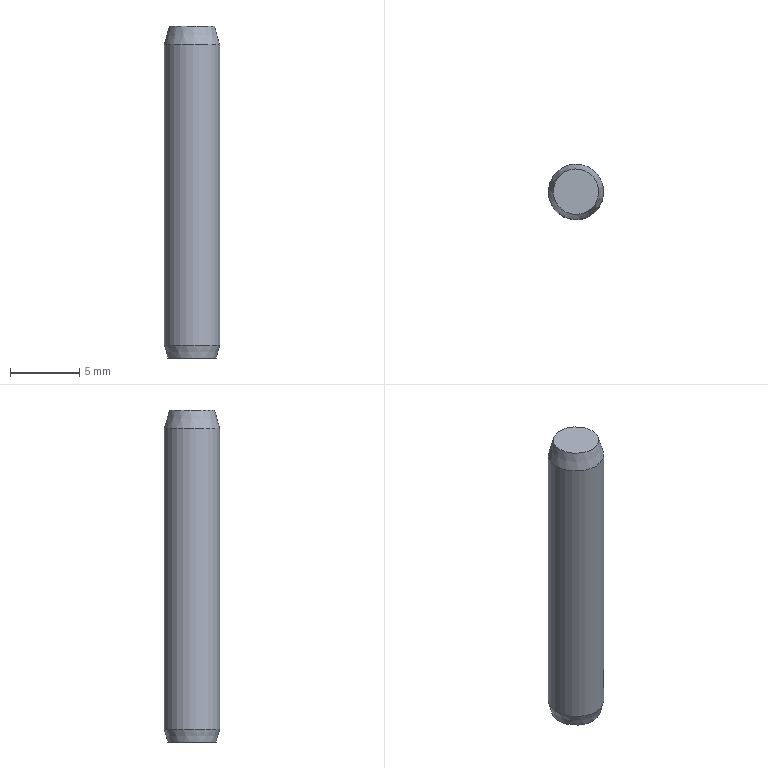Component | NX | 15_T120_1_M4X24_THREADED_DOWEL_PIN_2 | 1 solid | 9 faces | box 4 x 4 x 24 mm | volume 280 mm3 | cone 4 | cylinder 3 | plane 2 | commonest cylinder face diameters 4 x1 1.22 x1 2.3 x1
STEP:
#1=CARTESIAN_POINT('',(0.,0.,0.));
#2=DIRECTION('',(0.,0.,1.));
#3=DIRECTION('',(1.,0.,0.));
#4=AXIS2_PLACEMENT_3D('',#1,#2,#3);
#5=CARTESIAN_POINT('',(19.847,13.766,0.9317));
#6=VERTEX_POINT('',#5);
#7=CARTESIAN_POINT('',(18.,13.,0.9317));
#8=DIRECTION('',(0.,0.,1.));
#9=DIRECTION('',(0.9237,0.383,0.));
#10=AXIS2_PLACEMENT_3D('',#7,#8,#9);
#11=CIRCLE('',#10,2.);
#12=CARTESIAN_POINT('',(18.,13.,0.2588));
#13=DIRECTION('',(0.,0.,1.));
#14=DIRECTION('',(0.9237,0.383,0.));
#15=AXIS2_PLACEMENT_3D('',#12,#13,#14);
#16=CONICAL_SURFACE('',#15,1.82,0.2618);
#17=CARTESIAN_POINT('',(0.,0.6728));
#18=DIRECTION('',(1.,0.));
#19=VECTOR('',#18,1.);
#20=LINE('',#17,#19);
#21=(GEOMETRIC_REPRESENTATION_CONTEXT(2)PARAMETRIC_REPRESENTATION_CONTEXT()REPRESENTATION_CONTEXT('',''));
#22=DEFINITIONAL_REPRESENTATION('',(#20),#21);
#23=PCURVE('',#16,#22);
#24=CARTESIAN_POINT('',(18.,13.,-0.));
#25=DIRECTION('',(0.,0.,1.));
#26=DIRECTION('',(0.9237,0.383,0.));
#27=AXIS2_PLACEMENT_3D('',#24,#25,#26);
#28=CYLINDRICAL_SURFACE('',#27,2.);
#29=CARTESIAN_POINT('',(0.,0.9317));
#30=DIRECTION('',(1.,0.));
#31=VECTOR('',#30,1.);
#32=LINE('',#29,#31);
#33=(GEOMETRIC_REPRESENTATION_CONTEXT(2)PARAMETRIC_REPRESENTATION_CONTEXT()REPRESENTATION_CONTEXT('',''));
#34=DEFINITIONAL_REPRESENTATION('',(#32),#33);
#35=PCURVE('',#28,#34);
#36=SURFACE_CURVE('',#11,(#23,#35),.PCURVE_S1.);
#37=EDGE_CURVE('',#6,#6,#36,.T.);
#38=ORIENTED_EDGE('',*,*,#37,.F.);
#39=CARTESIAN_POINT('',(19.617,13.67,-0.));
#40=VERTEX_POINT('',#39);
#41=CARTESIAN_POINT('',(19.617,13.67,-0.));
#42=CARTESIAN_POINT('',(19.847,13.766,0.9317));
#43=B_SPLINE_CURVE_WITH_KNOTS('',1,(#41,#42),.UNSPECIFIED.,.F.,.F.,(2,2),(-0.2679,0.6966),.PIECEWISE_BEZIER_KNOTS.);
#44=CARTESIAN_POINT('',(0.,0.));
#45=DIRECTION('',(0.,1.));
#46=VECTOR('',#45,1.);
#47=LINE('',#44,#46);
#48=(GEOMETRIC_REPRESENTATION_CONTEXT(2)PARAMETRIC_REPRESENTATION_CONTEXT()REPRESENTATION_CONTEXT('',''));
#49=DEFINITIONAL_REPRESENTATION('',(#47),#48);
#50=PCURVE('',#16,#49);
#51=CARTESIAN_POINT('',(6.283,0.));
#52=DIRECTION('',(0.,1.));
#53=VECTOR('',#52,1.);
#54=LINE('',#51,#53);
#55=(GEOMETRIC_REPRESENTATION_CONTEXT(2)PARAMETRIC_REPRESENTATION_CONTEXT()REPRESENTATION_CONTEXT('',''));
#56=DEFINITIONAL_REPRESENTATION('',(#54),#55);
#57=PCURVE('',#16,#56);
#58=SEAM_CURVE('',#43,(#50,#57),.PCURVE_S1.);
#59=EDGE_CURVE('',#40,#6,#58,.T.);
#60=ORIENTED_EDGE('',*,*,#59,.F.);
#61=CARTESIAN_POINT('',(18.,13.,-0.));
#62=DIRECTION('',(0.,0.,1.));
#63=DIRECTION('',(0.9237,0.383,0.));
#64=AXIS2_PLACEMENT_3D('',#61,#62,#63);
#65=CIRCLE('',#64,1.75);
#66=CARTESIAN_POINT('',(0.,-0.2588));
#67=DIRECTION('',(1.,0.));
#68=VECTOR('',#67,1.);
#69=LINE('',#66,#68);
#70=(GEOMETRIC_REPRESENTATION_CONTEXT(2)PARAMETRIC_REPRESENTATION_CONTEXT()REPRESENTATION_CONTEXT('',''));
#71=DEFINITIONAL_REPRESENTATION('',(#69),#70);
#72=PCURVE('',#16,#71);
#73=CARTESIAN_POINT('',(17.176,14.986,-0.));
#74=DIRECTION('',(0.,0.,1.));
#75=DIRECTION('',(0.9237,0.383,0.));
#76=AXIS2_PLACEMENT_3D('',#73,#74,#75);
#77=PLANE('',#76);
#78=CARTESIAN_POINT('',(0.,-2.15));
#79=DIRECTION('',(1.,-0.));
#80=AXIS2_PLACEMENT_2D('',#78,#79);
#81=CIRCLE('',#80,1.75);
#82=(GEOMETRIC_REPRESENTATION_CONTEXT(2)PARAMETRIC_REPRESENTATION_CONTEXT()REPRESENTATION_CONTEXT('',''));
#83=DEFINITIONAL_REPRESENTATION('',(#81),#82);
#84=PCURVE('',#77,#83);
#85=SURFACE_CURVE('',#65,(#72,#84),.PCURVE_S1.);
#86=EDGE_CURVE('',#40,#40,#85,.T.);
#87=ORIENTED_EDGE('',*,*,#86,.T.);
#88=ORIENTED_EDGE('',*,*,#59,.T.);
#89=EDGE_LOOP('',(#38,#60,#87,#88));
#90=FACE_BOUND('',#89,.T.);
#91=ADVANCED_FACE('',(#90),#16,.T.);
#92=CARTESIAN_POINT('',(19.847,13.766,22.668));
#93=VERTEX_POINT('',#92);
#94=CARTESIAN_POINT('',(16.153,12.234,22.668));
#95=VERTEX_POINT('',#94);
#96=CARTESIAN_POINT('',(18.,13.,22.668));
#97=DIRECTION('',(0.,0.,1.));
#98=DIRECTION('',(-0.9237,-0.383,0.));
#99=AXIS2_PLACEMENT_3D('',#96,#97,#98);
#100=CIRCLE('',#99,2.);
#101=CARTESIAN_POINT('',(-3.142,22.668));
#102=DIRECTION('',(1.,0.));
#103=VECTOR('',#102,1.);
#104=LINE('',#101,#103);
#105=(GEOMETRIC_REPRESENTATION_CONTEXT(2)PARAMETRIC_REPRESENTATION_CONTEXT()REPRESENTATION_CONTEXT('',''));
#106=DEFINITIONAL_REPRESENTATION('',(#104),#105);
#107=PCURVE('',#28,#106);
#108=CARTESIAN_POINT('',(18.,13.,22.541));
#109=DIRECTION('',(0.,0.,-1.));
#110=DIRECTION('',(-0.9237,-0.383,0.));
#111=AXIS2_PLACEMENT_3D('',#108,#109,#110);
#112=CONICAL_SURFACE('',#111,2.034,0.2618);
#113=CARTESIAN_POINT('',(6.283,-0.1272));
#114=DIRECTION('',(-1.,0.));
#115=VECTOR('',#114,1.);
#116=LINE('',#113,#115);
#117=(GEOMETRIC_REPRESENTATION_CONTEXT(2)PARAMETRIC_REPRESENTATION_CONTEXT()REPRESENTATION_CONTEXT('',''));
#118=DEFINITIONAL_REPRESENTATION('',(#116),#117);
#119=PCURVE('',#112,#118);
#120=SURFACE_CURVE('',#100,(#107,#119),.PCURVE_S1.);
#121=EDGE_CURVE('',#93,#95,#120,.T.);
#122=ORIENTED_EDGE('',*,*,#121,.F.);
#123=CARTESIAN_POINT('',(19.847,13.766,0.9317));
#124=CARTESIAN_POINT('',(19.847,13.766,22.668));
#125=B_SPLINE_CURVE_WITH_KNOTS('',1,(#123,#124),.UNSPECIFIED.,.F.,.F.,(2,2),(0.9317,22.668),.PIECEWISE_BEZIER_KNOTS.);
#126=CARTESIAN_POINT('',(0.,0.));
#127=DIRECTION('',(0.,1.));
#128=VECTOR('',#127,1.);
#129=LINE('',#126,#128);
#130=(GEOMETRIC_REPRESENTATION_CONTEXT(2)PARAMETRIC_REPRESENTATION_CONTEXT()REPRESENTATION_CONTEXT('',''));
#131=DEFINITIONAL_REPRESENTATION('',(#129),#130);
#132=PCURVE('',#28,#131);
#133=CARTESIAN_POINT('',(6.283,0.));
#134=DIRECTION('',(0.,1.));
#135=VECTOR('',#134,1.);
#136=LINE('',#133,#135);
#137=(GEOMETRIC_REPRESENTATION_CONTEXT(2)PARAMETRIC_REPRESENTATION_CONTEXT()REPRESENTATION_CONTEXT('',''));
#138=DEFINITIONAL_REPRESENTATION('',(#136),#137);
#139=PCURVE('',#28,#138);
#140=SEAM_CURVE('',#125,(#132,#139),.PCURVE_S1.);
#141=EDGE_CURVE('',#6,#93,#140,.T.);
#142=ORIENTED_EDGE('',*,*,#141,.F.);
#143=ORIENTED_EDGE('',*,*,#37,.T.);
#144=ORIENTED_EDGE('',*,*,#141,.T.);
#145=CARTESIAN_POINT('',(18.,13.,22.668));
#146=DIRECTION('',(0.,0.,1.));
#147=DIRECTION('',(-0.9237,-0.383,0.));
#148=AXIS2_PLACEMENT_3D('',#145,#146,#147);
#149=CIRCLE('',#148,2.);
#150=CARTESIAN_POINT('',(3.142,22.668));
#151=DIRECTION('',(1.,0.));
#152=VECTOR('',#151,1.);
#153=LINE('',#150,#152);
#154=(GEOMETRIC_REPRESENTATION_CONTEXT(2)PARAMETRIC_REPRESENTATION_CONTEXT()REPRESENTATION_CONTEXT('',''));
#155=DEFINITIONAL_REPRESENTATION('',(#153),#154);
#156=PCURVE('',#28,#155);
#157=CARTESIAN_POINT('',(6.283,-0.1272));
#158=DIRECTION('',(-1.,0.));
#159=VECTOR('',#158,1.);
#160=LINE('',#157,#159);
#161=(GEOMETRIC_REPRESENTATION_CONTEXT(2)PARAMETRIC_REPRESENTATION_CONTEXT()REPRESENTATION_CONTEXT('',''));
#162=DEFINITIONAL_REPRESENTATION('',(#160),#161);
#163=PCURVE('',#112,#162);
#164=SURFACE_CURVE('',#149,(#156,#163),.PCURVE_S1.);
#165=EDGE_CURVE('',#95,#93,#164,.T.);
#166=ORIENTED_EDGE('',*,*,#165,.F.);
#167=EDGE_LOOP('',(#122,#142,#143,#144,#166));
#168=FACE_BOUND('',#167,.T.);
#169=ADVANCED_FACE('',(#168),#28,.T.);
#170=CARTESIAN_POINT('',(16.482,12.371,24.));
#171=VERTEX_POINT('',#170);
#172=CARTESIAN_POINT('',(18.,13.,24.));
#173=DIRECTION('',(0.,0.,1.));
#174=DIRECTION('',(-0.9237,-0.383,0.));
#175=AXIS2_PLACEMENT_3D('',#172,#173,#174);
#176=CIRCLE('',#175,1.643);
#177=CARTESIAN_POINT('',(6.283,-1.459));
#178=DIRECTION('',(-1.,0.));
#179=VECTOR('',#178,1.);
#180=LINE('',#177,#179);
#181=(GEOMETRIC_REPRESENTATION_CONTEXT(2)PARAMETRIC_REPRESENTATION_CONTEXT()REPRESENTATION_CONTEXT('',''));
#182=DEFINITIONAL_REPRESENTATION('',(#180),#181);
#183=PCURVE('',#112,#182);
#184=CARTESIAN_POINT('',(16.974,15.474,24.));
#185=DIRECTION('',(0.,0.,-1.));
#186=DIRECTION('',(-0.9237,-0.383,0.));
#187=AXIS2_PLACEMENT_3D('',#184,#185,#186);
#188=PLANE('',#187);
#189=CARTESIAN_POINT('',(1.643,-2.678));
#190=CARTESIAN_POINT('',(1.643,-5.525));
#191=CARTESIAN_POINT('',(-0.8216,-4.102));
#192=CARTESIAN_POINT('',(-3.286,-2.678));
#193=CARTESIAN_POINT('',(-0.8216,-1.255));
#194=CARTESIAN_POINT('',(1.643,0.1676));
#195=CARTESIAN_POINT('',(1.643,-2.678));
#196=(BOUNDED_CURVE()B_SPLINE_CURVE(2,(#189,#190,#191,#192,#193,#194,#195),.UNSPECIFIED.,.T.,.F.)B_SPLINE_CURVE_WITH_KNOTS((1,2,2,2,2,1),(-2.094,0.,2.094,4.189,6.283,8.378),.UNSPECIFIED.)CURVE()GEOMETRIC_REPRESENTATION_ITEM()RATIONAL_B_SPLINE_CURVE((1.,0.5,1.,0.5,1.,0.5,1.))REPRESENTATION_ITEM(''));
#197=(GEOMETRIC_REPRESENTATION_CONTEXT(2)PARAMETRIC_REPRESENTATION_CONTEXT()REPRESENTATION_CONTEXT('',''));
#198=DEFINITIONAL_REPRESENTATION('',(#196),#197);
#199=PCURVE('',#188,#198);
#200=SURFACE_CURVE('',#176,(#183,#199),.PCURVE_S1.);
#201=EDGE_CURVE('',#171,#171,#200,.T.);
#202=ORIENTED_EDGE('',*,*,#201,.F.);
#203=CARTESIAN_POINT('',(16.482,12.371,24.));
#204=CARTESIAN_POINT('',(16.153,12.234,22.668));
#205=B_SPLINE_CURVE_WITH_KNOTS('',1,(#203,#204),.UNSPECIFIED.,.F.,.F.,(2,2),(-1.51,-0.1317),.PIECEWISE_BEZIER_KNOTS.);
#206=CARTESIAN_POINT('',(6.283,0.));
#207=DIRECTION('',(0.,1.));
#208=VECTOR('',#207,1.);
#209=LINE('',#206,#208);
#210=(GEOMETRIC_REPRESENTATION_CONTEXT(2)PARAMETRIC_REPRESENTATION_CONTEXT()REPRESENTATION_CONTEXT('',''));
#211=DEFINITIONAL_REPRESENTATION('',(#209),#210);
#212=PCURVE('',#112,#211);
#213=CARTESIAN_POINT('',(0.,0.));
#214=DIRECTION('',(0.,1.));
#215=VECTOR('',#214,1.);
#216=LINE('',#213,#215);
#217=(GEOMETRIC_REPRESENTATION_CONTEXT(2)PARAMETRIC_REPRESENTATION_CONTEXT()REPRESENTATION_CONTEXT('',''));
#218=DEFINITIONAL_REPRESENTATION('',(#216),#217);
#219=PCURVE('',#112,#218);
#220=SEAM_CURVE('',#205,(#212,#219),.PCURVE_S1.);
#221=EDGE_CURVE('',#171,#95,#220,.T.);
#222=ORIENTED_EDGE('',*,*,#221,.T.);
#223=ORIENTED_EDGE('',*,*,#165,.T.);
#224=ORIENTED_EDGE('',*,*,#121,.T.);
#225=ORIENTED_EDGE('',*,*,#221,.F.);
#226=EDGE_LOOP('',(#202,#222,#223,#224,#225));
#227=FACE_BOUND('',#226,.T.);
#228=ADVANCED_FACE('',(#227),#112,.T.);
#229=ORIENTED_EDGE('',*,*,#201,.T.);
#230=EDGE_LOOP('',(#229));
#231=FACE_BOUND('',#230,.T.);
#232=ADVANCED_FACE('',(#231),#188,.F.);
#233=CARTESIAN_POINT('',(17.437,12.766,10.577));
#234=VERTEX_POINT('',#233);
#235=CARTESIAN_POINT('',(18.,13.,10.577));
#236=DIRECTION('',(0.,0.,1.));
#237=DIRECTION('',(-0.9237,-0.383,0.));
#238=AXIS2_PLACEMENT_3D('',#235,#236,#237);
#239=CIRCLE('',#238,0.61);
#240=CARTESIAN_POINT('',(18.,13.,10.93));
#241=DIRECTION('',(0.,0.,-1.));
#242=DIRECTION('',(-0.9237,-0.383,0.));
#243=AXIS2_PLACEMENT_3D('',#240,#241,#242);
#244=CONICAL_SURFACE('',#243,0.,1.047);
#245=CARTESIAN_POINT('',(6.283,0.3522));
#246=DIRECTION('',(-1.,-0.));
#247=VECTOR('',#246,1.);
#248=LINE('',#245,#247);
#249=(GEOMETRIC_REPRESENTATION_CONTEXT(2)PARAMETRIC_REPRESENTATION_CONTEXT()REPRESENTATION_CONTEXT('',''));
#250=DEFINITIONAL_REPRESENTATION('',(#248),#249);
#251=PCURVE('',#244,#250);
#252=CARTESIAN_POINT('',(18.,13.,-0.));
#253=DIRECTION('',(0.,0.,1.));
#254=DIRECTION('',(0.9237,0.383,0.));
#255=AXIS2_PLACEMENT_3D('',#252,#253,#254);
#256=CYLINDRICAL_SURFACE('',#255,0.61);
#257=CARTESIAN_POINT('',(3.142,10.577));
#258=DIRECTION('',(1.,0.));
#259=VECTOR('',#258,1.);
#260=LINE('',#257,#259);
#261=(GEOMETRIC_REPRESENTATION_CONTEXT(2)PARAMETRIC_REPRESENTATION_CONTEXT()REPRESENTATION_CONTEXT('',''));
#262=DEFINITIONAL_REPRESENTATION('',(#260),#261);
#263=PCURVE('',#256,#262);
#264=SURFACE_CURVE('',#239,(#251,#263),.PCURVE_S1.);
#265=EDGE_CURVE('',#234,#234,#264,.T.);
#266=ORIENTED_EDGE('',*,*,#265,.T.);
#267=CARTESIAN_POINT('',(18.,13.,10.93));
#268=VERTEX_POINT('',#267);
#269=CARTESIAN_POINT('',(18.,13.,10.93));
#270=CARTESIAN_POINT('',(17.437,12.766,10.577));
#271=B_SPLINE_CURVE_WITH_KNOTS('',1,(#269,#270),.UNSPECIFIED.,.F.,.F.,(2,2),(-0.,0.7044),.PIECEWISE_BEZIER_KNOTS.);
#272=CARTESIAN_POINT('',(0.,0.));
#273=DIRECTION('',(0.,1.));
#274=VECTOR('',#273,1.);
#275=LINE('',#272,#274);
#276=(GEOMETRIC_REPRESENTATION_CONTEXT(2)PARAMETRIC_REPRESENTATION_CONTEXT()REPRESENTATION_CONTEXT('',''));
#277=DEFINITIONAL_REPRESENTATION('',(#275),#276);
#278=PCURVE('',#244,#277);
#279=CARTESIAN_POINT('',(6.283,0.));
#280=DIRECTION('',(0.,1.));
#281=VECTOR('',#280,1.);
#282=LINE('',#279,#281);
#283=(GEOMETRIC_REPRESENTATION_CONTEXT(2)PARAMETRIC_REPRESENTATION_CONTEXT()REPRESENTATION_CONTEXT('',''));
#284=DEFINITIONAL_REPRESENTATION('',(#282),#283);
#285=PCURVE('',#244,#284);
#286=SEAM_CURVE('',#271,(#278,#285),.PCURVE_S1.);
#287=EDGE_CURVE('',#268,#234,#286,.T.);
#288=ORIENTED_EDGE('',*,*,#287,.F.);
#289=ORIENTED_EDGE('',*,*,#287,.T.);
#290=EDGE_LOOP('',(#266,#288,#289));
#291=FACE_BOUND('',#290,.F.);
#292=ADVANCED_FACE('',(#291),#244,.F.);
#293=CARTESIAN_POINT('',(17.437,12.766,1.889));
#294=VERTEX_POINT('',#293);
#295=CARTESIAN_POINT('',(18.,13.,1.889));
#296=DIRECTION('',(0.,0.,1.));
#297=DIRECTION('',(-0.9237,-0.383,0.));
#298=AXIS2_PLACEMENT_3D('',#295,#296,#297);
#299=CIRCLE('',#298,0.61);
#300=CARTESIAN_POINT('',(3.142,1.889));
#301=DIRECTION('',(1.,0.));
#302=VECTOR('',#301,1.);
#303=LINE('',#300,#302);
#304=(GEOMETRIC_REPRESENTATION_CONTEXT(2)PARAMETRIC_REPRESENTATION_CONTEXT()REPRESENTATION_CONTEXT('',''));
#305=DEFINITIONAL_REPRESENTATION('',(#303),#304);
#306=PCURVE('',#256,#305);
#307=CARTESIAN_POINT('',(18.,13.,1.312));
#308=DIRECTION('',(0.,0.,-1.));
#309=DIRECTION('',(-0.9237,-0.383,0.));
#310=AXIS2_PLACEMENT_3D('',#307,#308,#309);
#311=CONICAL_SURFACE('',#310,1.61,1.047);
#312=CARTESIAN_POINT('',(6.283,-0.5774));
#313=DIRECTION('',(-1.,0.));
#314=VECTOR('',#313,1.);
#315=LINE('',#312,#314);
#316=(GEOMETRIC_REPRESENTATION_CONTEXT(2)PARAMETRIC_REPRESENTATION_CONTEXT()REPRESENTATION_CONTEXT('',''));
#317=DEFINITIONAL_REPRESENTATION('',(#315),#316);
#318=PCURVE('',#311,#317);
#319=SURFACE_CURVE('',#299,(#306,#318),.PCURVE_S1.);
#320=EDGE_CURVE('',#294,#294,#319,.T.);
#321=ORIENTED_EDGE('',*,*,#320,.T.);
#322=CARTESIAN_POINT('',(17.437,12.766,1.889));
#323=CARTESIAN_POINT('',(17.437,12.766,10.577));
#324=B_SPLINE_CURVE_WITH_KNOTS('',1,(#322,#323),.UNSPECIFIED.,.F.,.F.,(2,2),(1.889,10.577),.PIECEWISE_BEZIER_KNOTS.);
#325=CARTESIAN_POINT('',(9.425,0.));
#326=DIRECTION('',(0.,1.));
#327=VECTOR('',#326,1.);
#328=LINE('',#325,#327);
#329=(GEOMETRIC_REPRESENTATION_CONTEXT(2)PARAMETRIC_REPRESENTATION_CONTEXT()REPRESENTATION_CONTEXT('',''));
#330=DEFINITIONAL_REPRESENTATION('',(#328),#329);
#331=PCURVE('',#256,#330);
#332=CARTESIAN_POINT('',(3.142,0.));
#333=DIRECTION('',(0.,1.));
#334=VECTOR('',#333,1.);
#335=LINE('',#332,#334);
#336=(GEOMETRIC_REPRESENTATION_CONTEXT(2)PARAMETRIC_REPRESENTATION_CONTEXT()REPRESENTATION_CONTEXT('',''));
#337=DEFINITIONAL_REPRESENTATION('',(#335),#336);
#338=PCURVE('',#256,#337);
#339=SEAM_CURVE('',#324,(#331,#338),.PCURVE_S1.);
#340=EDGE_CURVE('',#294,#234,#339,.T.);
#341=ORIENTED_EDGE('',*,*,#340,.T.);
#342=ORIENTED_EDGE('',*,*,#265,.F.);
#343=ORIENTED_EDGE('',*,*,#340,.F.);
#344=EDGE_LOOP('',(#321,#341,#342,#343));
#345=FACE_BOUND('',#344,.F.);
#346=ADVANCED_FACE('',(#345),#256,.F.);
#347=CARTESIAN_POINT('',(16.938,12.559,1.577));
#348=VERTEX_POINT('',#347);
#349=CARTESIAN_POINT('',(19.062,13.441,1.577));
#350=VERTEX_POINT('',#349);
#351=CARTESIAN_POINT('',(18.,13.,1.577));
#352=DIRECTION('',(0.,0.,1.));
#353=DIRECTION('',(-0.9237,-0.383,0.));
#354=AXIS2_PLACEMENT_3D('',#351,#352,#353);
#355=CIRCLE('',#354,1.15);
#356=CARTESIAN_POINT('',(6.283,-0.2656));
#357=DIRECTION('',(-1.,0.));
#358=VECTOR('',#357,1.);
#359=LINE('',#356,#358);
#360=(GEOMETRIC_REPRESENTATION_CONTEXT(2)PARAMETRIC_REPRESENTATION_CONTEXT()REPRESENTATION_CONTEXT('',''));
#361=DEFINITIONAL_REPRESENTATION('',(#359),#360);
#362=PCURVE('',#311,#361);
#363=CARTESIAN_POINT('',(18.,13.,-0.));
#364=DIRECTION('',(0.,0.,1.));
#365=DIRECTION('',(0.9237,0.383,0.));
#366=AXIS2_PLACEMENT_3D('',#363,#364,#365);
#367=CYLINDRICAL_SURFACE('',#366,1.15);
#368=CARTESIAN_POINT('',(3.142,1.577));
#369=DIRECTION('',(1.,0.));
#370=VECTOR('',#369,1.);
#371=LINE('',#368,#370);
#372=(GEOMETRIC_REPRESENTATION_CONTEXT(2)PARAMETRIC_REPRESENTATION_CONTEXT()REPRESENTATION_CONTEXT('',''));
#373=DEFINITIONAL_REPRESENTATION('',(#371),#372);
#374=PCURVE('',#367,#373);
#375=SURFACE_CURVE('',#355,(#362,#374),.PCURVE_S1.);
#376=EDGE_CURVE('',#348,#350,#375,.T.);
#377=ORIENTED_EDGE('',*,*,#376,.T.);
#378=CARTESIAN_POINT('',(18.,13.,1.577));
#379=DIRECTION('',(0.,0.,1.));
#380=DIRECTION('',(-0.9237,-0.383,0.));
#381=AXIS2_PLACEMENT_3D('',#378,#379,#380);
#382=CIRCLE('',#381,1.15);
#383=CARTESIAN_POINT('',(6.283,-0.2656));
#384=DIRECTION('',(-1.,0.));
#385=VECTOR('',#384,1.);
#386=LINE('',#383,#385);
#387=(GEOMETRIC_REPRESENTATION_CONTEXT(2)PARAMETRIC_REPRESENTATION_CONTEXT()REPRESENTATION_CONTEXT('',''));
#388=DEFINITIONAL_REPRESENTATION('',(#386),#387);
#389=PCURVE('',#311,#388);
#390=CARTESIAN_POINT('',(-3.142,1.577));
#391=DIRECTION('',(1.,0.));
#392=VECTOR('',#391,1.);
#393=LINE('',#390,#392);
#394=(GEOMETRIC_REPRESENTATION_CONTEXT(2)PARAMETRIC_REPRESENTATION_CONTEXT()REPRESENTATION_CONTEXT('',''));
#395=DEFINITIONAL_REPRESENTATION('',(#393),#394);
#396=PCURVE('',#367,#395);
#397=SURFACE_CURVE('',#382,(#389,#396),.PCURVE_S1.);
#398=EDGE_CURVE('',#350,#348,#397,.T.);
#399=ORIENTED_EDGE('',*,*,#398,.T.);
#400=CARTESIAN_POINT('',(17.437,12.766,1.889));
#401=CARTESIAN_POINT('',(16.938,12.559,1.577));
#402=B_SPLINE_CURVE_WITH_KNOTS('',1,(#400,#401),.UNSPECIFIED.,.F.,.F.,(2,2),(-1.155,-0.5312),.PIECEWISE_BEZIER_KNOTS.);
#403=CARTESIAN_POINT('',(0.,0.));
#404=DIRECTION('',(0.,1.));
#405=VECTOR('',#404,1.);
#406=LINE('',#403,#405);
#407=(GEOMETRIC_REPRESENTATION_CONTEXT(2)PARAMETRIC_REPRESENTATION_CONTEXT()REPRESENTATION_CONTEXT('',''));
#408=DEFINITIONAL_REPRESENTATION('',(#406),#407);
#409=PCURVE('',#311,#408);
#410=CARTESIAN_POINT('',(6.283,0.));
#411=DIRECTION('',(0.,1.));
#412=VECTOR('',#411,1.);
#413=LINE('',#410,#412);
#414=(GEOMETRIC_REPRESENTATION_CONTEXT(2)PARAMETRIC_REPRESENTATION_CONTEXT()REPRESENTATION_CONTEXT('',''));
#415=DEFINITIONAL_REPRESENTATION('',(#413),#414);
#416=PCURVE('',#311,#415);
#417=SEAM_CURVE('',#402,(#409,#416),.PCURVE_S1.);
#418=EDGE_CURVE('',#294,#348,#417,.T.);
#419=ORIENTED_EDGE('',*,*,#418,.F.);
#420=ORIENTED_EDGE('',*,*,#320,.F.);
#421=ORIENTED_EDGE('',*,*,#418,.T.);
#422=EDGE_LOOP('',(#377,#399,#419,#420,#421));
#423=FACE_BOUND('',#422,.F.);
#424=ADVANCED_FACE('',(#423),#311,.F.);
#425=CARTESIAN_POINT('',(19.062,13.441,-0.));
#426=VERTEX_POINT('',#425);
#427=CARTESIAN_POINT('',(18.,13.,-0.));
#428=DIRECTION('',(0.,0.,1.));
#429=DIRECTION('',(0.9237,0.383,0.));
#430=AXIS2_PLACEMENT_3D('',#427,#428,#429);
#431=CIRCLE('',#430,1.15);
#432=CARTESIAN_POINT('',(0.,0.));
#433=DIRECTION('',(1.,0.));
#434=VECTOR('',#433,1.);
#435=LINE('',#432,#434);
#436=(GEOMETRIC_REPRESENTATION_CONTEXT(2)PARAMETRIC_REPRESENTATION_CONTEXT()REPRESENTATION_CONTEXT('',''));
#437=DEFINITIONAL_REPRESENTATION('',(#435),#436);
#438=PCURVE('',#367,#437);
#439=CARTESIAN_POINT('',(0.,-2.15));
#440=DIRECTION('',(1.,0.));
#441=AXIS2_PLACEMENT_2D('',#439,#440);
#442=CIRCLE('',#441,1.15);
#443=(GEOMETRIC_REPRESENTATION_CONTEXT(2)PARAMETRIC_REPRESENTATION_CONTEXT()REPRESENTATION_CONTEXT('',''));
#444=DEFINITIONAL_REPRESENTATION('',(#442),#443);
#445=PCURVE('',#77,#444);
#446=SURFACE_CURVE('',#431,(#438,#445),.PCURVE_S1.);
#447=EDGE_CURVE('',#426,#426,#446,.T.);
#448=ORIENTED_EDGE('',*,*,#447,.T.);
#449=CARTESIAN_POINT('',(19.062,13.441,-0.));
#450=CARTESIAN_POINT('',(19.062,13.441,1.577));
#451=B_SPLINE_CURVE_WITH_KNOTS('',1,(#449,#450),.UNSPECIFIED.,.F.,.F.,(2,2),(0.,1.577),.PIECEWISE_BEZIER_KNOTS.);
#452=CARTESIAN_POINT('',(6.283,0.));
#453=DIRECTION('',(0.,1.));
#454=VECTOR('',#453,1.);
#455=LINE('',#452,#454);
#456=(GEOMETRIC_REPRESENTATION_CONTEXT(2)PARAMETRIC_REPRESENTATION_CONTEXT()REPRESENTATION_CONTEXT('',''));
#457=DEFINITIONAL_REPRESENTATION('',(#455),#456);
#458=PCURVE('',#367,#457);
#459=CARTESIAN_POINT('',(0.,0.));
#460=DIRECTION('',(0.,1.));
#461=VECTOR('',#460,1.);
#462=LINE('',#459,#461);
#463=(GEOMETRIC_REPRESENTATION_CONTEXT(2)PARAMETRIC_REPRESENTATION_CONTEXT()REPRESENTATION_CONTEXT('',''));
#464=DEFINITIONAL_REPRESENTATION('',(#462),#463);
#465=PCURVE('',#367,#464);
#466=SEAM_CURVE('',#451,(#458,#465),.PCURVE_S1.);
#467=EDGE_CURVE('',#426,#350,#466,.T.);
#468=ORIENTED_EDGE('',*,*,#467,.T.);
#469=ORIENTED_EDGE('',*,*,#376,.F.);
#470=ORIENTED_EDGE('',*,*,#398,.F.);
#471=ORIENTED_EDGE('',*,*,#467,.F.);
#472=EDGE_LOOP('',(#448,#468,#469,#470,#471));
#473=FACE_BOUND('',#472,.F.);
#474=ADVANCED_FACE('',(#473),#367,.F.);
#475=ORIENTED_EDGE('',*,*,#86,.F.);
#476=EDGE_LOOP('',(#475));
#477=FACE_BOUND('',#476,.T.);
#478=ORIENTED_EDGE('',*,*,#447,.T.);
#479=EDGE_LOOP('',(#478));
#480=FACE_BOUND('',#479,.T.);
#481=ADVANCED_FACE('',(#477,#480),#77,.F.);
#482=CLOSED_SHELL('',(#91,#169,#228,#232,#292,#346,#424,#474,#481));
#483=MANIFOLD_SOLID_BREP('',#482);
#484=(LENGTH_UNIT()NAMED_UNIT(*)SI_UNIT(.MILLI.,.METRE.));
#485=UNCERTAINTY_MEASURE_WITH_UNIT(LENGTH_MEASURE(0.00001),#484,'','');
#486=(NAMED_UNIT(*)PLANE_ANGLE_UNIT()SI_UNIT($,.RADIAN.));
#487=(NAMED_UNIT(*)SI_UNIT($,.STERADIAN.)SOLID_ANGLE_UNIT());
#488=(GEOMETRIC_REPRESENTATION_CONTEXT(3)GLOBAL_UNCERTAINTY_ASSIGNED_CONTEXT((#485))GLOBAL_UNIT_ASSIGNED_CONTEXT((#484,#486,#487))REPRESENTATION_CONTEXT('',''));
#489=ADVANCED_BREP_SHAPE_REPRESENTATION('',(#4,#483),#488);